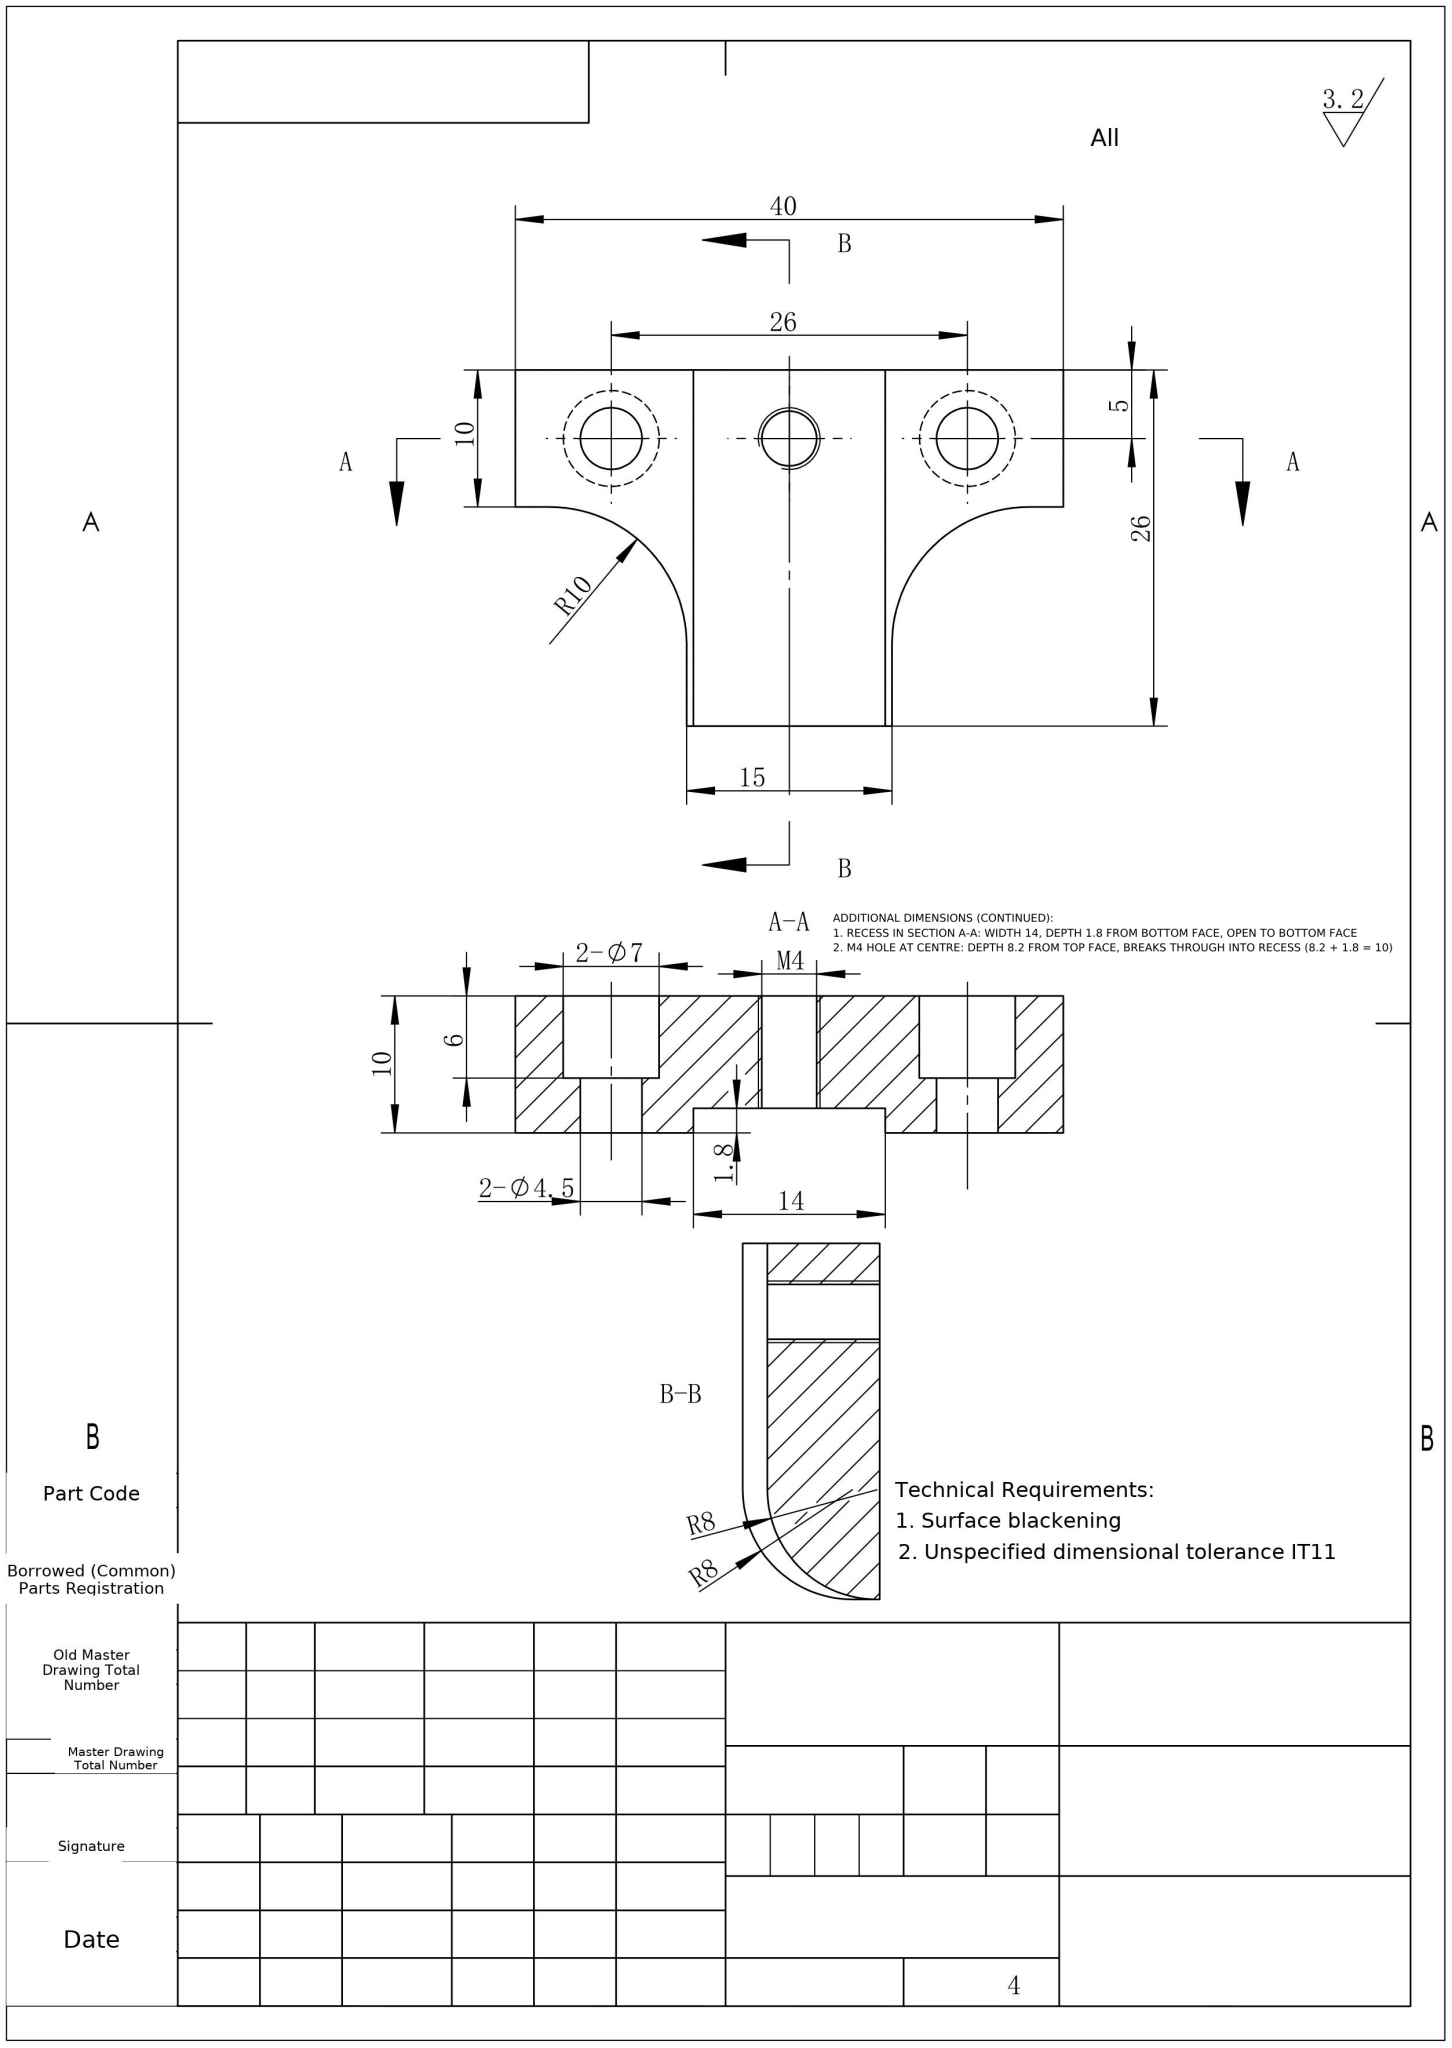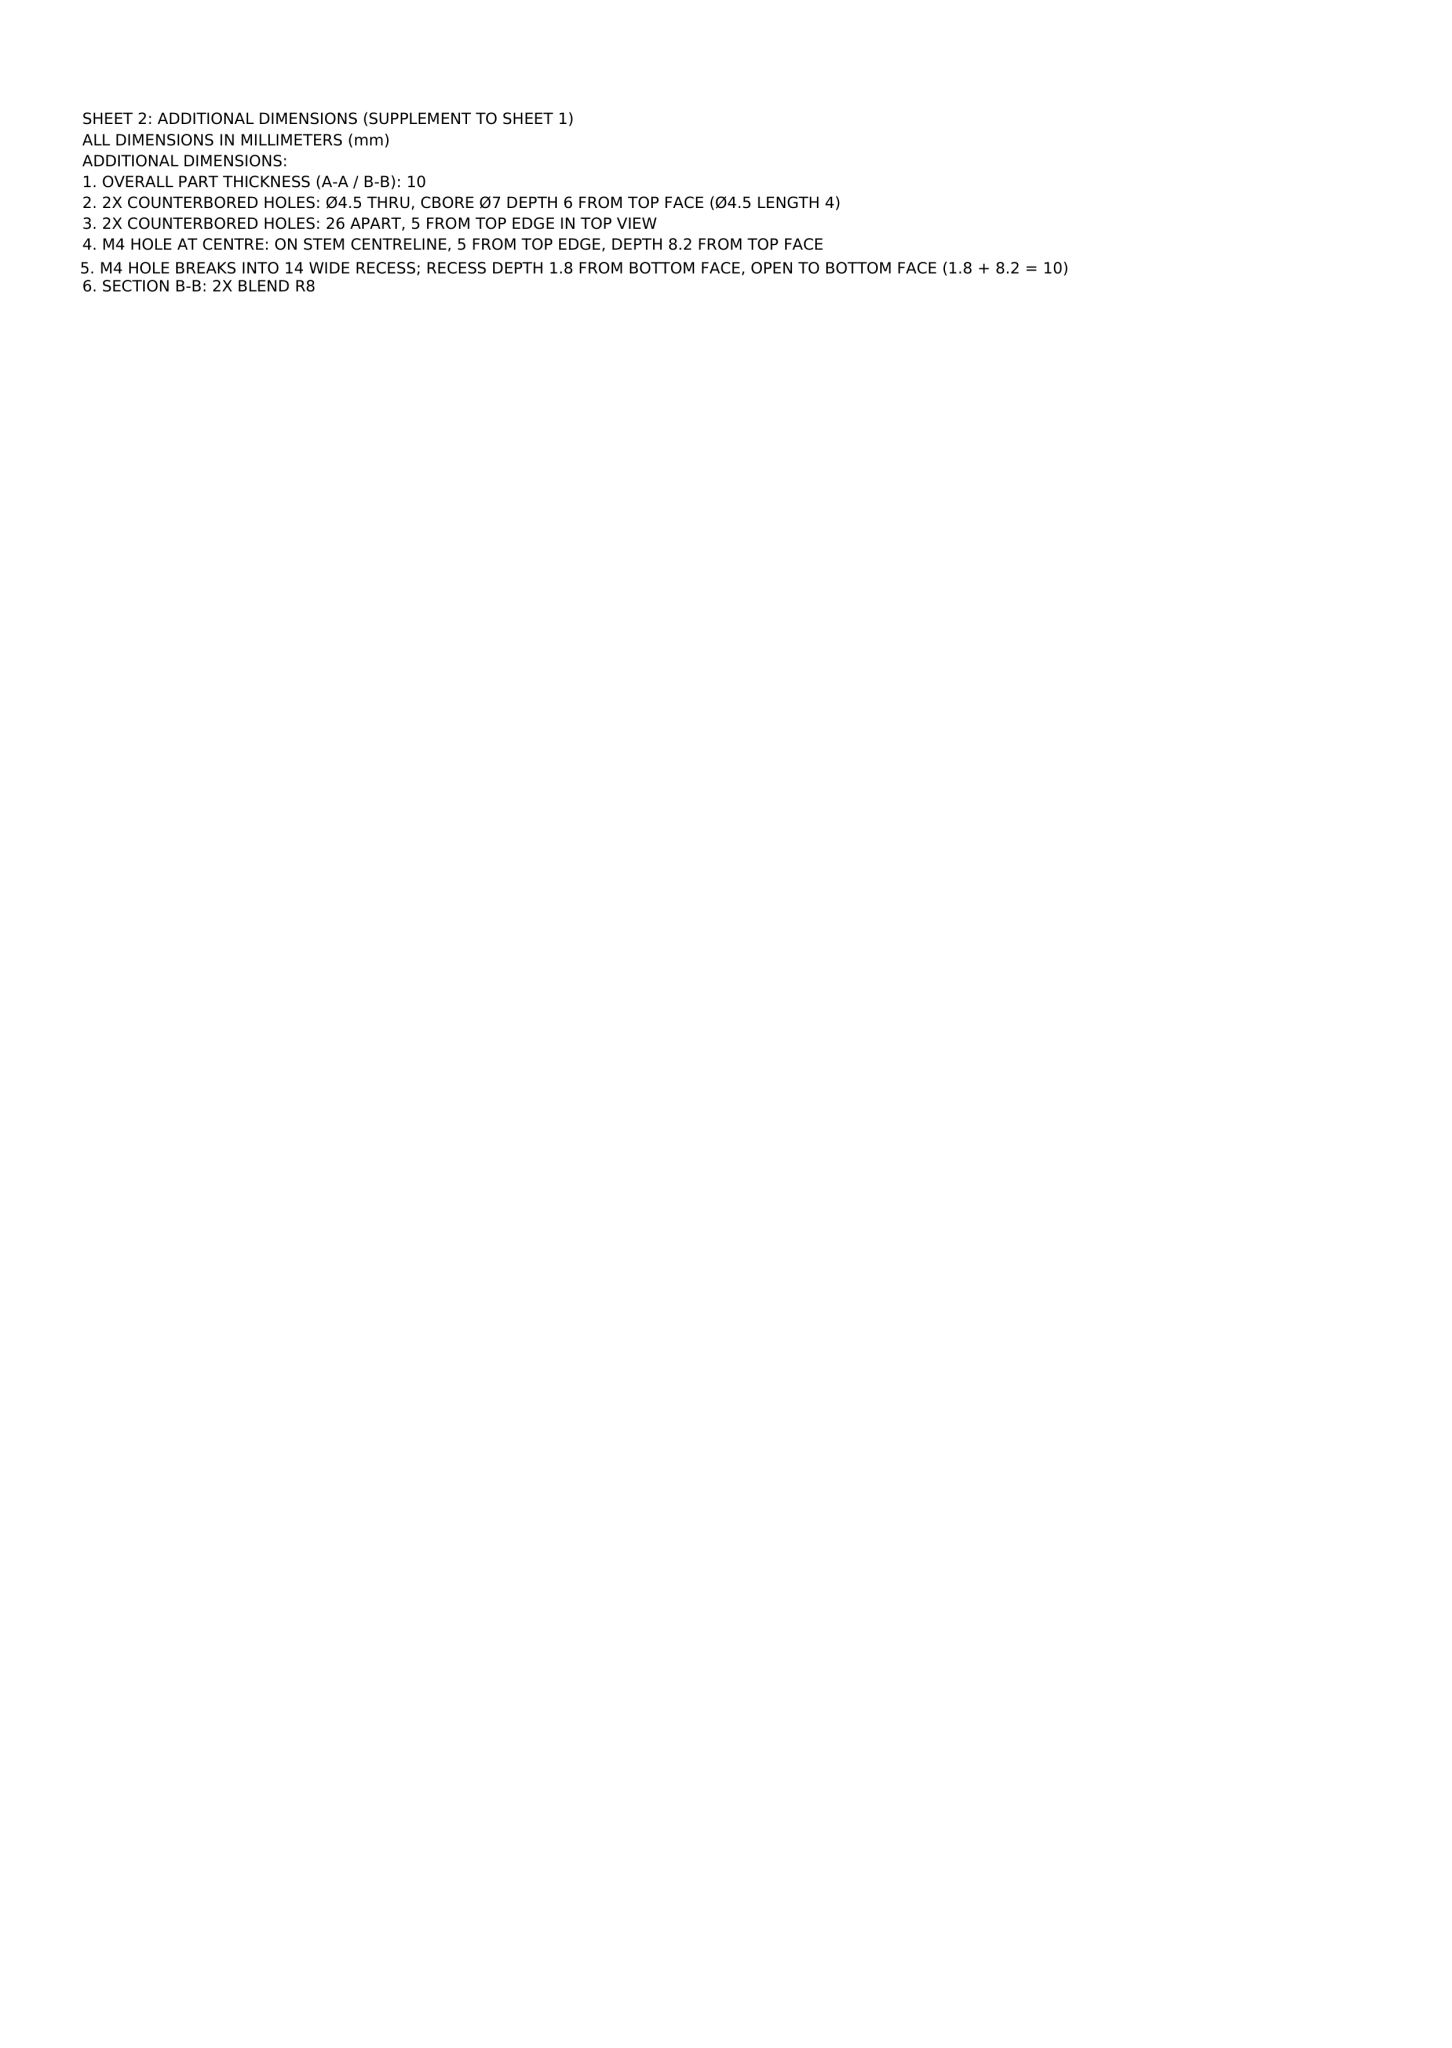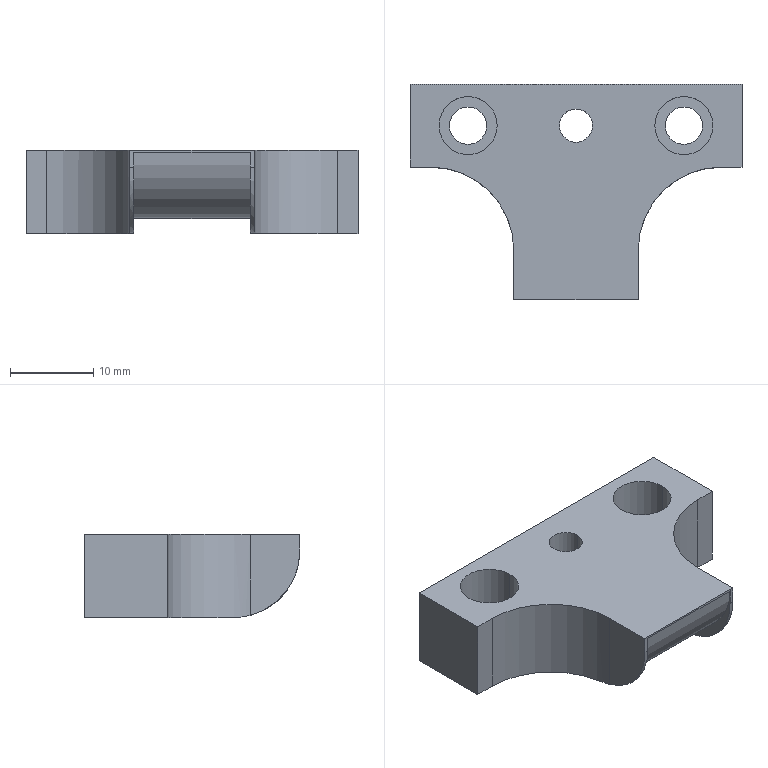Part | NX | mm | 1 solid | 31 faces | box 40 x 26 x 10 mm | volume 5276 mm3 | plane 16 | cylinder 15 | commonest cylinder face diameters 7 x4 4.5 x4 16 x3 4 x2 20 x2